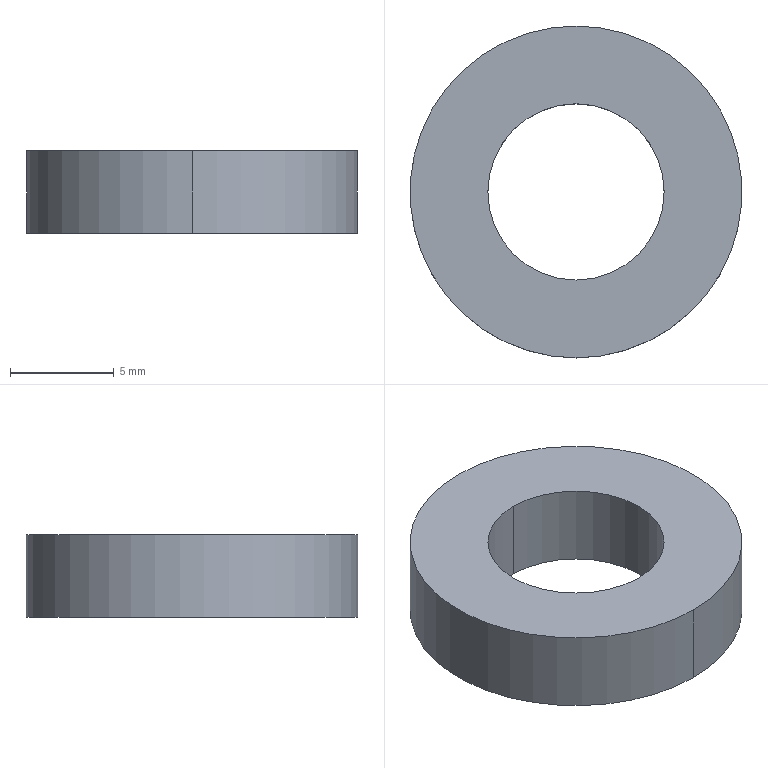Component | SolidWorks | Part1342542-2 | 1 solid | 6 faces | box 16 x 16 x 4 mm | volume 577 mm3 | cylinder 4 | plane 2 | commonest cylinder face diameters 8.5 x2 16 x2
build123d program:
from build123d import *

# Parameters (mm, degrees)
SKETCH1_R           = 8
SKETCH1_R_2         = 4.25
BOSS_EXTRUDE1_DEPTH = 4


with BuildPart() as part:
    # Sketch1 → Boss-Extrude1 (new body)
    with BuildSketch(Plane(origin=(0, 0, 0), x_dir=(1, 0, 0), z_dir=(0, 1, 0))):
        with Locations(Location((0, 0, 0), (0, 0, 270))):
            Circle(SKETCH1_R)
        with Locations(Location((0, 0, 0), (0, 0, 270))):
            Circle(SKETCH1_R_2, mode=Mode.SUBTRACT)
    extrude(amount=BOSS_EXTRUDE1_DEPTH)


solid = part.part

# Placed as in the assembly
solid = solid.moved(Location((935.266, 337.75, -259.945), (90, 0, 0)))
STEP:
#1=COLOUR_RGB('',0.7922,0.8196,0.9333);
#2=FILL_AREA_STYLE_COLOUR('',#1);
#3=FILL_AREA_STYLE('',(#2));
#4=SURFACE_STYLE_FILL_AREA(#3);
#5=SURFACE_SIDE_STYLE('',(#4));
#6=SURFACE_STYLE_USAGE(.BOTH.,#5);
#7=PRESENTATION_STYLE_ASSIGNMENT((#6));
#8=CARTESIAN_POINT('',(36.822,13.13,-10.234));
#9=VERTEX_POINT('',#8);
#10=CARTESIAN_POINT('',(36.822,13.465,-10.234));
#11=VERTEX_POINT('',#10);
#12=CARTESIAN_POINT('',(36.822,13.297,-10.234));
#13=DIRECTION('',(-0.00002551,-0.,-1.));
#14=DIRECTION('',(-0.00002551,1.,0.));
#15=AXIS2_PLACEMENT_3D('',#12,#13,#14);
#16=CIRCLE('',#15,0.1673);
#17=EDGE_CURVE('',#9,#11,#16,.T.);
#18=ORIENTED_EDGE('',*,*,#17,.T.);
#19=CARTESIAN_POINT('',(36.822,13.465,-10.077));
#20=VERTEX_POINT('',#19);
#21=CARTESIAN_POINT('',(36.822,13.465,-10.234));
#22=DIRECTION('',(0.00002551,0.,1.));
#23=VECTOR('',#22,39.37);
#24=LINE('',#21,#23);
#25=EDGE_CURVE('',#11,#20,#24,.T.);
#26=ORIENTED_EDGE('',*,*,#25,.T.);
#27=CARTESIAN_POINT('',(36.822,13.13,-10.077));
#28=VERTEX_POINT('',#27);
#29=CARTESIAN_POINT('',(36.822,13.297,-10.077));
#30=DIRECTION('',(-0.00002551,-0.,-1.));
#31=DIRECTION('',(-0.00002551,1.,0.));
#32=AXIS2_PLACEMENT_3D('',#29,#30,#31);
#33=CIRCLE('',#32,0.1673);
#34=EDGE_CURVE('',#28,#20,#33,.T.);
#35=ORIENTED_EDGE('',*,*,#34,.F.);
#36=CARTESIAN_POINT('',(36.822,13.13,-10.234));
#37=DIRECTION('',(0.00002551,0.,1.));
#38=VECTOR('',#37,39.37);
#39=LINE('',#36,#38);
#40=EDGE_CURVE('',#9,#28,#39,.T.);
#41=ORIENTED_EDGE('',*,*,#40,.F.);
#42=EDGE_LOOP('',(#18,#26,#35,#41));
#43=FACE_OUTER_BOUND('',#42,.T.);
#44=CARTESIAN_POINT('',(36.822,13.297,-10.234));
#45=DIRECTION('',(0.00002551,0.,1.));
#46=DIRECTION('',(0.00002551,-1.,-0.));
#47=AXIS2_PLACEMENT_3D('',#44,#45,#46);
#48=CYLINDRICAL_SURFACE('',#47,0.1673);
#49=ADVANCED_FACE('',(#43),#48,.F.);
#50=CARTESIAN_POINT('',(36.822,13.612,-10.234));
#51=VERTEX_POINT('',#50);
#52=CARTESIAN_POINT('',(36.822,12.982,-10.234));
#53=VERTEX_POINT('',#52);
#54=CARTESIAN_POINT('',(36.822,13.297,-10.234));
#55=DIRECTION('',(-0.00002551,-0.,-1.));
#56=DIRECTION('',(-0.00002551,1.,0.));
#57=AXIS2_PLACEMENT_3D('',#54,#55,#56);
#58=CIRCLE('',#57,0.315);
#59=EDGE_CURVE('',#51,#53,#58,.T.);
#60=ORIENTED_EDGE('',*,*,#59,.F.);
#61=CARTESIAN_POINT('',(36.822,13.612,-10.077));
#62=VERTEX_POINT('',#61);
#63=CARTESIAN_POINT('',(36.822,13.612,-10.234));
#64=DIRECTION('',(0.00002551,0.,1.));
#65=VECTOR('',#64,39.37);
#66=LINE('',#63,#65);
#67=EDGE_CURVE('',#51,#62,#66,.T.);
#68=ORIENTED_EDGE('',*,*,#67,.T.);
#69=CARTESIAN_POINT('',(36.822,12.982,-10.077));
#70=VERTEX_POINT('',#69);
#71=CARTESIAN_POINT('',(36.822,13.297,-10.077));
#72=DIRECTION('',(-0.00002551,-0.,-1.));
#73=DIRECTION('',(-0.00002551,1.,0.));
#74=AXIS2_PLACEMENT_3D('',#71,#72,#73);
#75=CIRCLE('',#74,0.315);
#76=EDGE_CURVE('',#62,#70,#75,.T.);
#77=ORIENTED_EDGE('',*,*,#76,.T.);
#78=CARTESIAN_POINT('',(36.822,12.982,-10.234));
#79=DIRECTION('',(0.00002551,0.,1.));
#80=VECTOR('',#79,39.37);
#81=LINE('',#78,#80);
#82=EDGE_CURVE('',#53,#70,#81,.T.);
#83=ORIENTED_EDGE('',*,*,#82,.F.);
#84=EDGE_LOOP('',(#60,#68,#77,#83));
#85=FACE_OUTER_BOUND('',#84,.T.);
#86=CARTESIAN_POINT('',(36.822,13.297,-10.234));
#87=DIRECTION('',(0.00002551,0.,1.));
#88=DIRECTION('',(0.00002551,-1.,-0.));
#89=AXIS2_PLACEMENT_3D('',#86,#87,#88);
#90=CYLINDRICAL_SURFACE('',#89,0.315);
#91=ADVANCED_FACE('',(#85),#90,.T.);
#92=CARTESIAN_POINT('',(36.822,13.297,-10.234));
#93=DIRECTION('',(-0.00002551,-0.,-1.));
#94=DIRECTION('',(-0.00002551,1.,0.));
#95=AXIS2_PLACEMENT_3D('',#92,#93,#94);
#96=CIRCLE('',#95,0.315);
#97=EDGE_CURVE('',#53,#51,#96,.T.);
#98=ORIENTED_EDGE('',*,*,#97,.T.);
#99=ORIENTED_EDGE('',*,*,#59,.T.);
#100=EDGE_LOOP('',(#98,#99));
#101=FACE_OUTER_BOUND('',#100,.T.);
#102=ORIENTED_EDGE('',*,*,#17,.F.);
#103=CARTESIAN_POINT('',(36.822,13.297,-10.234));
#104=DIRECTION('',(-0.00002551,-0.,-1.));
#105=DIRECTION('',(-0.00002551,1.,0.));
#106=AXIS2_PLACEMENT_3D('',#103,#104,#105);
#107=CIRCLE('',#106,0.1673);
#108=EDGE_CURVE('',#11,#9,#107,.T.);
#109=ORIENTED_EDGE('',*,*,#108,.F.);
#110=EDGE_LOOP('',(#102,#109));
#111=FACE_BOUND('',#110,.T.);
#112=CARTESIAN_POINT('',(36.822,13.297,-10.234));
#113=DIRECTION('',(-0.00002551,-0.,-1.));
#114=DIRECTION('',(-0.00002551,1.,0.));
#115=AXIS2_PLACEMENT_3D('',#112,#113,#114);
#116=PLANE('',#115);
#117=ADVANCED_FACE('',(#101,#111),#116,.T.);
#118=CARTESIAN_POINT('',(36.822,13.297,-10.077));
#119=DIRECTION('',(-0.00002551,-0.,-1.));
#120=DIRECTION('',(-0.00002551,1.,0.));
#121=AXIS2_PLACEMENT_3D('',#118,#119,#120);
#122=CIRCLE('',#121,0.315);
#123=EDGE_CURVE('',#70,#62,#122,.T.);
#124=ORIENTED_EDGE('',*,*,#123,.F.);
#125=ORIENTED_EDGE('',*,*,#76,.F.);
#126=EDGE_LOOP('',(#124,#125));
#127=FACE_OUTER_BOUND('',#126,.T.);
#128=ORIENTED_EDGE('',*,*,#34,.T.);
#129=CARTESIAN_POINT('',(36.822,13.297,-10.077));
#130=DIRECTION('',(-0.00002551,-0.,-1.));
#131=DIRECTION('',(-0.00002551,1.,0.));
#132=AXIS2_PLACEMENT_3D('',#129,#130,#131);
#133=CIRCLE('',#132,0.1673);
#134=EDGE_CURVE('',#20,#28,#133,.T.);
#135=ORIENTED_EDGE('',*,*,#134,.T.);
#136=EDGE_LOOP('',(#128,#135));
#137=FACE_BOUND('',#136,.T.);
#138=CARTESIAN_POINT('',(36.822,13.297,-10.077));
#139=DIRECTION('',(-0.00002551,-0.,-1.));
#140=DIRECTION('',(-0.00002551,1.,0.));
#141=AXIS2_PLACEMENT_3D('',#138,#139,#140);
#142=PLANE('',#141);
#143=ADVANCED_FACE('',(#127,#137),#142,.F.);
#144=ORIENTED_EDGE('',*,*,#67,.F.);
#145=ORIENTED_EDGE('',*,*,#97,.F.);
#146=ORIENTED_EDGE('',*,*,#82,.T.);
#147=ORIENTED_EDGE('',*,*,#123,.T.);
#148=EDGE_LOOP('',(#144,#145,#146,#147));
#149=FACE_OUTER_BOUND('',#148,.T.);
#150=CARTESIAN_POINT('',(36.822,13.297,-10.234));
#151=DIRECTION('',(0.00002551,0.,1.));
#152=DIRECTION('',(0.00002551,-1.,-0.));
#153=AXIS2_PLACEMENT_3D('',#150,#151,#152);
#154=CYLINDRICAL_SURFACE('',#153,0.315);
#155=ADVANCED_FACE('',(#149),#154,.T.);
#156=ORIENTED_EDGE('',*,*,#25,.F.);
#157=ORIENTED_EDGE('',*,*,#108,.T.);
#158=ORIENTED_EDGE('',*,*,#40,.T.);
#159=ORIENTED_EDGE('',*,*,#134,.F.);
#160=EDGE_LOOP('',(#156,#157,#158,#159));
#161=FACE_OUTER_BOUND('',#160,.T.);
#162=CARTESIAN_POINT('',(36.822,13.297,-10.234));
#163=DIRECTION('',(0.00002551,0.,1.));
#164=DIRECTION('',(0.00002551,-1.,-0.));
#165=AXIS2_PLACEMENT_3D('',#162,#163,#164);
#166=CYLINDRICAL_SURFACE('',#165,0.1673);
#167=ADVANCED_FACE('',(#161),#166,.F.);
#168=CLOSED_SHELL('',(#49,#91,#117,#143,#155,#167));
#169=MANIFOLD_SOLID_BREP('',#168);
#170=STYLED_ITEM('',(#7),#169);
#171=PRESENTATION_LAYER_ASSIGNMENT('','',(#170));
#172=CARTESIAN_POINT('',(0.,0.,0.));
#173=DIRECTION('',(0.,0.,1.));
#174=DIRECTION('',(1.,0.,0.));
#175=AXIS2_PLACEMENT_3D('',#172,#173,#174);
#176=(LENGTH_UNIT()NAMED_UNIT(*)SI_UNIT($,.METRE.));
#177=LENGTH_MEASURE_WITH_UNIT(LENGTH_MEASURE(0.0254),#176);
#178=DIMENSIONAL_EXPONENTS(1.,0.,0.,0.,0.,0.,0.);
#179=(CONVERSION_BASED_UNIT('',#177)LENGTH_UNIT()NAMED_UNIT(#178));
#180=UNCERTAINTY_MEASURE_WITH_UNIT(LENGTH_MEASURE(0.00001),#179,'','');
#181=(NAMED_UNIT(*)PLANE_ANGLE_UNIT()SI_UNIT($,.RADIAN.));
#182=(NAMED_UNIT(*)SI_UNIT($,.STERADIAN.)SOLID_ANGLE_UNIT());
#183=(GEOMETRIC_REPRESENTATION_CONTEXT(3)GLOBAL_UNCERTAINTY_ASSIGNED_CONTEXT((#180))GLOBAL_UNIT_ASSIGNED_CONTEXT((#179,#181,#182))REPRESENTATION_CONTEXT('',''));
#184=ADVANCED_BREP_SHAPE_REPRESENTATION('',(#169,#175),#183);
#185=(LENGTH_UNIT()NAMED_UNIT(*)SI_UNIT($,.METRE.));
#186=LENGTH_MEASURE_WITH_UNIT(LENGTH_MEASURE(0.0254),#185);
#187=DIMENSIONAL_EXPONENTS(1.,0.,0.,0.,0.,0.,0.);
#188=(CONVERSION_BASED_UNIT('',#186)LENGTH_UNIT()NAMED_UNIT(#187));
#189=UNCERTAINTY_MEASURE_WITH_UNIT(LENGTH_MEASURE(0.00001),#188,'','');
#190=(NAMED_UNIT(*)PLANE_ANGLE_UNIT()SI_UNIT($,.RADIAN.));
#191=(NAMED_UNIT(*)SI_UNIT($,.STERADIAN.)SOLID_ANGLE_UNIT());
#192=(GEOMETRIC_REPRESENTATION_CONTEXT(3)GLOBAL_UNCERTAINTY_ASSIGNED_CONTEXT((#189))GLOBAL_UNIT_ASSIGNED_CONTEXT((#188,#190,#191))REPRESENTATION_CONTEXT('',''));
#193=MECHANICAL_DESIGN_GEOMETRIC_PRESENTATION_REPRESENTATION('',(#170),#192);